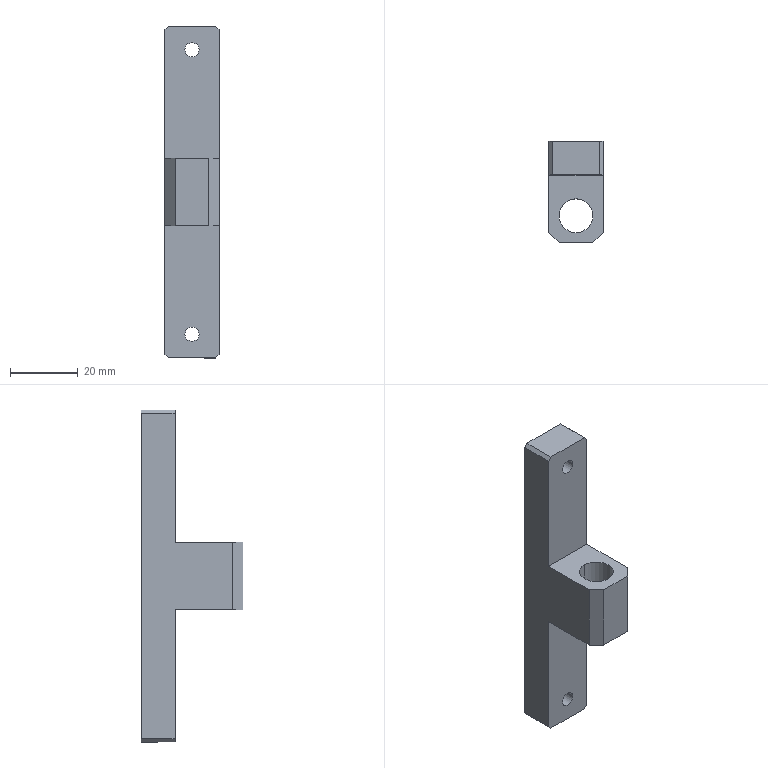Component | SolidWorks | XM-02-007A1-1 | 1 solid | 22 faces | box 16 x 30 x 98 mm | volume 20032 mm3 | plane 16 | cylinder 6 | commonest cylinder face diameters 4.2 x4 10 x2 | material 45#
build123d program:
from build123d import *

# Parameters (mm, degrees)
BOSS_EXTRUDE1_DEPTH = 16
SKETCH2_R           = 5
CUT_EXTRUDE1_DEPTH  = 69.096
M5_TAPPED_HOLE1_D   = 4.2
CHAMFER1_SIZE       = 3
CHAMFER2_SIZE       = 1


with BuildPart() as part:
    # Sketch1 → Boss-Extrude1 (new body)
    with BuildSketch(Plane.XY):
        Polygon((-10, 0), (10, 0), (10, 20), (49, 20), (49, 30), (-49, 30), (-49, 20), (-10, 20), align=None)
    extrude(amount=BOSS_EXTRUDE1_DEPTH)

    # Sketch2 → Cut-Extrude1 (cut, through all)
    with BuildSketch(Plane(origin=(10, 0, 0), x_dir=(0, 0, -1), z_dir=(1, 0, 0))):
        with Locations(Location((-8, 8, 0), (0, 0, 90))):
            Circle(SKETCH2_R)
    extrude(amount=-CUT_EXTRUDE1_DEPTH, mode=Mode.SUBTRACT)

    # M5 Tapped Hole1 (through all)
    with Locations(Plane(origin=(0, 30, 0), x_dir=(1, 0, 0), z_dir=(0, 1, 0))):
        with Locations((42, -8), (-42, -8)):
            Hole(M5_TAPPED_HOLE1_D / 2)

    # Chamfer1
    chamfer1_edges = [part.edges().sort_by_distance(p)[0] for p in [
        (0, 0, 0),
        (0, 0, 16),
    ]]
    chamfer(chamfer1_edges, length=CHAMFER1_SIZE)

    # Chamfer2
    chamfer2_edges = [part.edges().sort_by_distance(p)[0] for p in [
        (49, 25, 16),
        (-49, 25, 16),
        (-49, 25, 0),
        (49, 25, 0),
    ]]
    chamfer(chamfer2_edges, length=CHAMFER2_SIZE)


solid = part.part

# Placed as in the assembly
solid = solid.moved(Location((-5, -33, 0), (0, 90, 0)))
STEP:
#1=COLOUR_RGB('',0.7922,0.8196,0.9333);
#2=FILL_AREA_STYLE_COLOUR('',#1);
#3=FILL_AREA_STYLE('',(#2));
#4=SURFACE_STYLE_FILL_AREA(#3);
#5=SURFACE_SIDE_STYLE('',(#4));
#6=SURFACE_STYLE_USAGE(.BOTH.,#5);
#7=PRESENTATION_STYLE_ASSIGNMENT((#6));
#8=CARTESIAN_POINT('',(0.03543,-0.5118,-1.654));
#9=VERTEX_POINT('',#8);
#10=CARTESIAN_POINT('',(0.2008,-0.5118,-1.654));
#11=VERTEX_POINT('',#10);
#12=CARTESIAN_POINT('',(0.1181,-0.5118,-1.654));
#13=DIRECTION('',(-0.,1.,-0.));
#14=DIRECTION('',(0.,0.,1.));
#15=AXIS2_PLACEMENT_3D('',#12,#13,#14);
#16=CIRCLE('',#15,0.08268);
#17=EDGE_CURVE('',#9,#11,#16,.T.);
#18=ORIENTED_EDGE('',*,*,#17,.F.);
#19=CARTESIAN_POINT('',(0.03543,-0.1181,-1.654));
#20=VERTEX_POINT('',#19);
#21=CARTESIAN_POINT('',(0.03543,-0.1181,-1.654));
#22=DIRECTION('',(-0.,1.,-0.));
#23=VECTOR('',#22,39.37);
#24=LINE('',#21,#23);
#25=EDGE_CURVE('',#9,#20,#24,.T.);
#26=ORIENTED_EDGE('',*,*,#25,.T.);
#27=CARTESIAN_POINT('',(0.2008,-0.1181,-1.654));
#28=VERTEX_POINT('',#27);
#29=CARTESIAN_POINT('',(0.1181,-0.1181,-1.654));
#30=DIRECTION('',(-0.,1.,-0.));
#31=DIRECTION('',(1.,0.,0.));
#32=AXIS2_PLACEMENT_3D('',#29,#30,#31);
#33=CIRCLE('',#32,0.08268);
#34=EDGE_CURVE('',#20,#28,#33,.T.);
#35=ORIENTED_EDGE('',*,*,#34,.T.);
#36=CARTESIAN_POINT('',(0.2008,-0.1181,-1.654));
#37=DIRECTION('',(-0.,1.,-0.));
#38=VECTOR('',#37,39.37);
#39=LINE('',#36,#38);
#40=EDGE_CURVE('',#11,#28,#39,.T.);
#41=ORIENTED_EDGE('',*,*,#40,.F.);
#42=EDGE_LOOP('',(#18,#26,#35,#41));
#43=FACE_OUTER_BOUND('',#42,.T.);
#44=CARTESIAN_POINT('',(0.1181,-0.1181,-1.654));
#45=DIRECTION('',(-0.,1.,-0.));
#46=DIRECTION('',(1.,0.,0.));
#47=AXIS2_PLACEMENT_3D('',#44,#45,#46);
#48=CYLINDRICAL_SURFACE('',#47,0.08268);
#49=ADVANCED_FACE('',(#43),#48,.F.);
#50=CARTESIAN_POINT('',(0.03543,-0.5118,1.654));
#51=VERTEX_POINT('',#50);
#52=CARTESIAN_POINT('',(0.2008,-0.5118,1.654));
#53=VERTEX_POINT('',#52);
#54=CARTESIAN_POINT('',(0.1181,-0.5118,1.654));
#55=DIRECTION('',(-0.,1.,-0.));
#56=DIRECTION('',(0.,0.,1.));
#57=AXIS2_PLACEMENT_3D('',#54,#55,#56);
#58=CIRCLE('',#57,0.08268);
#59=EDGE_CURVE('',#51,#53,#58,.T.);
#60=ORIENTED_EDGE('',*,*,#59,.F.);
#61=CARTESIAN_POINT('',(0.03543,-0.1181,1.654));
#62=VERTEX_POINT('',#61);
#63=CARTESIAN_POINT('',(0.03543,-0.1181,1.654));
#64=DIRECTION('',(-0.,1.,-0.));
#65=VECTOR('',#64,39.37);
#66=LINE('',#63,#65);
#67=EDGE_CURVE('',#51,#62,#66,.T.);
#68=ORIENTED_EDGE('',*,*,#67,.T.);
#69=CARTESIAN_POINT('',(0.2008,-0.1181,1.654));
#70=VERTEX_POINT('',#69);
#71=CARTESIAN_POINT('',(0.1181,-0.1181,1.654));
#72=DIRECTION('',(-0.,1.,-0.));
#73=DIRECTION('',(1.,0.,0.));
#74=AXIS2_PLACEMENT_3D('',#71,#72,#73);
#75=CIRCLE('',#74,0.08268);
#76=EDGE_CURVE('',#62,#70,#75,.T.);
#77=ORIENTED_EDGE('',*,*,#76,.T.);
#78=CARTESIAN_POINT('',(0.2008,-0.1181,1.654));
#79=DIRECTION('',(-0.,1.,-0.));
#80=VECTOR('',#79,39.37);
#81=LINE('',#78,#80);
#82=EDGE_CURVE('',#53,#70,#81,.T.);
#83=ORIENTED_EDGE('',*,*,#82,.F.);
#84=EDGE_LOOP('',(#60,#68,#77,#83));
#85=FACE_OUTER_BOUND('',#84,.T.);
#86=CARTESIAN_POINT('',(0.1181,-0.1181,1.654));
#87=DIRECTION('',(-0.,1.,-0.));
#88=DIRECTION('',(1.,0.,0.));
#89=AXIS2_PLACEMENT_3D('',#86,#87,#88);
#90=CYLINDRICAL_SURFACE('',#89,0.08268);
#91=ADVANCED_FACE('',(#85),#90,.F.);
#92=CARTESIAN_POINT('',(0.1181,-1.181,0.3937));
#93=VERTEX_POINT('',#92);
#94=CARTESIAN_POINT('',(0.1181,-0.7874,0.3937));
#95=VERTEX_POINT('',#94);
#96=CARTESIAN_POINT('',(0.1181,-0.9843,0.3937));
#97=DIRECTION('',(-0.,-0.,-1.));
#98=DIRECTION('',(-1.,0.,0.));
#99=AXIS2_PLACEMENT_3D('',#96,#97,#98);
#100=CIRCLE('',#99,0.1969);
#101=EDGE_CURVE('',#93,#95,#100,.T.);
#102=ORIENTED_EDGE('',*,*,#101,.F.);
#103=CARTESIAN_POINT('',(0.1181,-1.181,-0.3937));
#104=VERTEX_POINT('',#103);
#105=CARTESIAN_POINT('',(0.1181,-1.181,1.929));
#106=DIRECTION('',(-0.,-0.,-1.));
#107=VECTOR('',#106,39.37);
#108=LINE('',#105,#107);
#109=EDGE_CURVE('',#93,#104,#108,.T.);
#110=ORIENTED_EDGE('',*,*,#109,.T.);
#111=CARTESIAN_POINT('',(0.1181,-0.7874,-0.3937));
#112=VERTEX_POINT('',#111);
#113=CARTESIAN_POINT('',(0.1181,-0.9843,-0.3937));
#114=DIRECTION('',(-0.,-0.,-1.));
#115=DIRECTION('',(-0.,1.,-0.));
#116=AXIS2_PLACEMENT_3D('',#113,#114,#115);
#117=CIRCLE('',#116,0.1969);
#118=EDGE_CURVE('',#104,#112,#117,.T.);
#119=ORIENTED_EDGE('',*,*,#118,.T.);
#120=CARTESIAN_POINT('',(0.1181,-0.7874,1.929));
#121=DIRECTION('',(-0.,-0.,-1.));
#122=VECTOR('',#121,39.37);
#123=LINE('',#120,#122);
#124=EDGE_CURVE('',#95,#112,#123,.T.);
#125=ORIENTED_EDGE('',*,*,#124,.F.);
#126=EDGE_LOOP('',(#102,#110,#119,#125));
#127=FACE_OUTER_BOUND('',#126,.T.);
#128=CARTESIAN_POINT('',(0.1181,-0.9843,1.929));
#129=DIRECTION('',(-0.,-0.,-1.));
#130=DIRECTION('',(-0.,1.,-0.));
#131=AXIS2_PLACEMENT_3D('',#128,#129,#130);
#132=CYLINDRICAL_SURFACE('',#131,0.1969);
#133=ADVANCED_FACE('',(#127),#132,.F.);
#134=CARTESIAN_POINT('',(0.1181,-0.9843,0.3937));
#135=DIRECTION('',(-0.,-0.,-1.));
#136=DIRECTION('',(-1.,0.,0.));
#137=AXIS2_PLACEMENT_3D('',#134,#135,#136);
#138=CIRCLE('',#137,0.1969);
#139=EDGE_CURVE('',#95,#93,#138,.T.);
#140=ORIENTED_EDGE('',*,*,#139,.T.);
#141=ORIENTED_EDGE('',*,*,#101,.T.);
#142=EDGE_LOOP('',(#140,#141));
#143=FACE_BOUND('',#142,.T.);
#144=CARTESIAN_POINT('',(0.315,-1.299,0.3937));
#145=VERTEX_POINT('',#144);
#146=CARTESIAN_POINT('',(-0.07874,-1.299,0.3937));
#147=VERTEX_POINT('',#146);
#148=CARTESIAN_POINT('',(0.4331,-1.299,0.3937));
#149=DIRECTION('',(-1.,-0.,0.));
#150=VECTOR('',#149,39.37);
#151=LINE('',#148,#150);
#152=EDGE_CURVE('',#145,#147,#151,.T.);
#153=ORIENTED_EDGE('',*,*,#152,.F.);
#154=CARTESIAN_POINT('',(0.4331,-1.181,0.3937));
#155=VERTEX_POINT('',#154);
#156=CARTESIAN_POINT('',(0.4331,-1.181,0.3937));
#157=DIRECTION('',(0.7071,0.7071,-0.));
#158=VECTOR('',#157,39.37);
#159=LINE('',#156,#158);
#160=EDGE_CURVE('',#145,#155,#159,.T.);
#161=ORIENTED_EDGE('',*,*,#160,.T.);
#162=CARTESIAN_POINT('',(0.4331,-0.5118,0.3937));
#163=VERTEX_POINT('',#162);
#164=CARTESIAN_POINT('',(0.4331,-0.5118,0.3937));
#165=DIRECTION('',(0.,-1.,0.));
#166=VECTOR('',#165,39.37);
#167=LINE('',#164,#166);
#168=EDGE_CURVE('',#163,#155,#167,.T.);
#169=ORIENTED_EDGE('',*,*,#168,.F.);
#170=CARTESIAN_POINT('',(-0.1969,-0.5118,0.3937));
#171=VERTEX_POINT('',#170);
#172=CARTESIAN_POINT('',(0.4331,-0.5118,0.3937));
#173=DIRECTION('',(-1.,-0.,0.));
#174=VECTOR('',#173,39.37);
#175=LINE('',#172,#174);
#176=EDGE_CURVE('',#163,#171,#175,.T.);
#177=ORIENTED_EDGE('',*,*,#176,.T.);
#178=CARTESIAN_POINT('',(-0.1969,-1.181,0.3937));
#179=VERTEX_POINT('',#178);
#180=CARTESIAN_POINT('',(-0.1969,-0.5118,0.3937));
#181=DIRECTION('',(0.,-1.,0.));
#182=VECTOR('',#181,39.37);
#183=LINE('',#180,#182);
#184=EDGE_CURVE('',#171,#179,#183,.T.);
#185=ORIENTED_EDGE('',*,*,#184,.T.);
#186=CARTESIAN_POINT('',(-0.07874,-1.299,0.3937));
#187=DIRECTION('',(0.7071,-0.7071,0.));
#188=VECTOR('',#187,39.37);
#189=LINE('',#186,#188);
#190=EDGE_CURVE('',#179,#147,#189,.T.);
#191=ORIENTED_EDGE('',*,*,#190,.T.);
#192=EDGE_LOOP('',(#153,#161,#169,#177,#185,#191));
#193=FACE_OUTER_BOUND('',#192,.T.);
#194=CARTESIAN_POINT('',(0.4331,-0.5118,0.3937));
#195=DIRECTION('',(-0.,-0.,-1.));
#196=DIRECTION('',(-1.,-0.,0.));
#197=AXIS2_PLACEMENT_3D('',#194,#195,#196);
#198=PLANE('',#197);
#199=ADVANCED_FACE('',(#143,#193),#198,.F.);
#200=CARTESIAN_POINT('',(0.315,-1.299,-0.3937));
#201=VERTEX_POINT('',#200);
#202=CARTESIAN_POINT('',(-0.07874,-1.299,-0.3937));
#203=VERTEX_POINT('',#202);
#204=CARTESIAN_POINT('',(0.4331,-1.299,-0.3937));
#205=DIRECTION('',(-1.,-0.,0.));
#206=VECTOR('',#205,39.37);
#207=LINE('',#204,#206);
#208=EDGE_CURVE('',#201,#203,#207,.T.);
#209=ORIENTED_EDGE('',*,*,#208,.F.);
#210=CARTESIAN_POINT('',(0.315,-1.299,0.3937));
#211=DIRECTION('',(0.,0.,1.));
#212=VECTOR('',#211,39.37);
#213=LINE('',#210,#212);
#214=EDGE_CURVE('',#201,#145,#213,.T.);
#215=ORIENTED_EDGE('',*,*,#214,.T.);
#216=ORIENTED_EDGE('',*,*,#152,.T.);
#217=CARTESIAN_POINT('',(-0.07874,-1.299,0.3937));
#218=DIRECTION('',(-0.,-0.,-1.));
#219=VECTOR('',#218,39.37);
#220=LINE('',#217,#219);
#221=EDGE_CURVE('',#147,#203,#220,.T.);
#222=ORIENTED_EDGE('',*,*,#221,.T.);
#223=EDGE_LOOP('',(#209,#215,#216,#222));
#224=FACE_OUTER_BOUND('',#223,.T.);
#225=CARTESIAN_POINT('',(0.4331,-1.299,0.3937));
#226=DIRECTION('',(-0.,1.,-0.));
#227=DIRECTION('',(0.,0.,1.));
#228=AXIS2_PLACEMENT_3D('',#225,#226,#227);
#229=PLANE('',#228);
#230=ADVANCED_FACE('',(#224),#229,.F.);
#231=CARTESIAN_POINT('',(0.1181,-0.9843,-0.3937));
#232=DIRECTION('',(-0.,-0.,-1.));
#233=DIRECTION('',(-0.,1.,-0.));
#234=AXIS2_PLACEMENT_3D('',#231,#232,#233);
#235=CIRCLE('',#234,0.1969);
#236=EDGE_CURVE('',#112,#104,#235,.T.);
#237=ORIENTED_EDGE('',*,*,#236,.F.);
#238=ORIENTED_EDGE('',*,*,#118,.F.);
#239=EDGE_LOOP('',(#237,#238));
#240=FACE_BOUND('',#239,.T.);
#241=CARTESIAN_POINT('',(0.4331,-1.181,-0.3937));
#242=VERTEX_POINT('',#241);
#243=CARTESIAN_POINT('',(0.4331,-0.5118,-0.3937));
#244=VERTEX_POINT('',#243);
#245=CARTESIAN_POINT('',(0.4331,-1.299,-0.3937));
#246=DIRECTION('',(-0.,1.,-0.));
#247=VECTOR('',#246,39.37);
#248=LINE('',#245,#247);
#249=EDGE_CURVE('',#242,#244,#248,.T.);
#250=ORIENTED_EDGE('',*,*,#249,.F.);
#251=CARTESIAN_POINT('',(0.4331,-1.181,-0.3937));
#252=DIRECTION('',(-0.7071,-0.7071,0.));
#253=VECTOR('',#252,39.37);
#254=LINE('',#251,#253);
#255=EDGE_CURVE('',#242,#201,#254,.T.);
#256=ORIENTED_EDGE('',*,*,#255,.T.);
#257=ORIENTED_EDGE('',*,*,#208,.T.);
#258=CARTESIAN_POINT('',(-0.1969,-1.181,-0.3937));
#259=VERTEX_POINT('',#258);
#260=CARTESIAN_POINT('',(-0.07874,-1.299,-0.3937));
#261=DIRECTION('',(-0.7071,0.7071,-0.));
#262=VECTOR('',#261,39.37);
#263=LINE('',#260,#262);
#264=EDGE_CURVE('',#203,#259,#263,.T.);
#265=ORIENTED_EDGE('',*,*,#264,.T.);
#266=CARTESIAN_POINT('',(-0.1969,-0.5118,-0.3937));
#267=VERTEX_POINT('',#266);
#268=CARTESIAN_POINT('',(-0.1969,-1.299,-0.3937));
#269=DIRECTION('',(-0.,1.,-0.));
#270=VECTOR('',#269,39.37);
#271=LINE('',#268,#270);
#272=EDGE_CURVE('',#259,#267,#271,.T.);
#273=ORIENTED_EDGE('',*,*,#272,.T.);
#274=CARTESIAN_POINT('',(0.4331,-0.5118,-0.3937));
#275=DIRECTION('',(-1.,-0.,0.));
#276=VECTOR('',#275,39.37);
#277=LINE('',#274,#276);
#278=EDGE_CURVE('',#244,#267,#277,.T.);
#279=ORIENTED_EDGE('',*,*,#278,.F.);
#280=EDGE_LOOP('',(#250,#256,#257,#265,#273,#279));
#281=FACE_OUTER_BOUND('',#280,.T.);
#282=CARTESIAN_POINT('',(0.4331,-1.299,-0.3937));
#283=DIRECTION('',(0.,0.,1.));
#284=DIRECTION('',(0.,-1.,0.));
#285=AXIS2_PLACEMENT_3D('',#282,#283,#284);
#286=PLANE('',#285);
#287=ADVANCED_FACE('',(#240,#281),#286,.F.);
#288=CARTESIAN_POINT('',(0.1181,-0.5118,-1.654));
#289=DIRECTION('',(-0.,1.,-0.));
#290=DIRECTION('',(0.,0.,1.));
#291=AXIS2_PLACEMENT_3D('',#288,#289,#290);
#292=CIRCLE('',#291,0.08268);
#293=EDGE_CURVE('',#11,#9,#292,.T.);
#294=ORIENTED_EDGE('',*,*,#293,.T.);
#295=ORIENTED_EDGE('',*,*,#17,.T.);
#296=EDGE_LOOP('',(#294,#295));
#297=FACE_BOUND('',#296,.T.);
#298=CARTESIAN_POINT('',(0.3937,-0.5118,-1.929));
#299=VERTEX_POINT('',#298);
#300=CARTESIAN_POINT('',(-0.1575,-0.5118,-1.929));
#301=VERTEX_POINT('',#300);
#302=CARTESIAN_POINT('',(0.4331,-0.5118,-1.929));
#303=DIRECTION('',(-1.,-0.,0.));
#304=VECTOR('',#303,39.37);
#305=LINE('',#302,#304);
#306=EDGE_CURVE('',#299,#301,#305,.T.);
#307=ORIENTED_EDGE('',*,*,#306,.F.);
#308=CARTESIAN_POINT('',(0.4331,-0.5118,-1.89));
#309=VERTEX_POINT('',#308);
#310=CARTESIAN_POINT('',(0.4331,-0.5118,-1.89));
#311=DIRECTION('',(0.7071,0.,0.7071));
#312=VECTOR('',#311,39.37);
#313=LINE('',#310,#312);
#314=EDGE_CURVE('',#299,#309,#313,.T.);
#315=ORIENTED_EDGE('',*,*,#314,.T.);
#316=CARTESIAN_POINT('',(0.4331,-0.5118,-0.3937));
#317=DIRECTION('',(-0.,-0.,-1.));
#318=VECTOR('',#317,39.37);
#319=LINE('',#316,#318);
#320=EDGE_CURVE('',#244,#309,#319,.T.);
#321=ORIENTED_EDGE('',*,*,#320,.F.);
#322=ORIENTED_EDGE('',*,*,#278,.T.);
#323=CARTESIAN_POINT('',(-0.1969,-0.5118,-1.89));
#324=VERTEX_POINT('',#323);
#325=CARTESIAN_POINT('',(-0.1969,-0.5118,-0.3937));
#326=DIRECTION('',(-0.,-0.,-1.));
#327=VECTOR('',#326,39.37);
#328=LINE('',#325,#327);
#329=EDGE_CURVE('',#267,#324,#328,.T.);
#330=ORIENTED_EDGE('',*,*,#329,.T.);
#331=CARTESIAN_POINT('',(-0.1575,-0.5118,-1.929));
#332=DIRECTION('',(0.7071,-0.,-0.7071));
#333=VECTOR('',#332,39.37);
#334=LINE('',#331,#333);
#335=EDGE_CURVE('',#324,#301,#334,.T.);
#336=ORIENTED_EDGE('',*,*,#335,.T.);
#337=EDGE_LOOP('',(#307,#315,#321,#322,#330,#336));
#338=FACE_OUTER_BOUND('',#337,.T.);
#339=CARTESIAN_POINT('',(0.4331,-0.5118,-0.3937));
#340=DIRECTION('',(-0.,1.,-0.));
#341=DIRECTION('',(0.,0.,1.));
#342=AXIS2_PLACEMENT_3D('',#339,#340,#341);
#343=PLANE('',#342);
#344=ADVANCED_FACE('',(#297,#338),#343,.F.);
#345=CARTESIAN_POINT('',(0.3937,-0.1181,-1.929));
#346=VERTEX_POINT('',#345);
#347=CARTESIAN_POINT('',(-0.1575,-0.1181,-1.929));
#348=VERTEX_POINT('',#347);
#349=CARTESIAN_POINT('',(0.4331,-0.1181,-1.929));
#350=DIRECTION('',(-1.,-0.,0.));
#351=VECTOR('',#350,39.37);
#352=LINE('',#349,#351);
#353=EDGE_CURVE('',#346,#348,#352,.T.);
#354=ORIENTED_EDGE('',*,*,#353,.F.);
#355=CARTESIAN_POINT('',(0.3937,-0.5118,-1.929));
#356=DIRECTION('',(0.,-1.,0.));
#357=VECTOR('',#356,39.37);
#358=LINE('',#355,#357);
#359=EDGE_CURVE('',#346,#299,#358,.T.);
#360=ORIENTED_EDGE('',*,*,#359,.T.);
#361=ORIENTED_EDGE('',*,*,#306,.T.);
#362=CARTESIAN_POINT('',(-0.1575,-0.5118,-1.929));
#363=DIRECTION('',(-0.,1.,-0.));
#364=VECTOR('',#363,39.37);
#365=LINE('',#362,#364);
#366=EDGE_CURVE('',#301,#348,#365,.T.);
#367=ORIENTED_EDGE('',*,*,#366,.T.);
#368=EDGE_LOOP('',(#354,#360,#361,#367));
#369=FACE_OUTER_BOUND('',#368,.T.);
#370=CARTESIAN_POINT('',(0.4331,-0.5118,-1.929));
#371=DIRECTION('',(0.,0.,1.));
#372=DIRECTION('',(1.,0.,-0.));
#373=AXIS2_PLACEMENT_3D('',#370,#371,#372);
#374=PLANE('',#373);
#375=ADVANCED_FACE('',(#369),#374,.F.);
#376=CARTESIAN_POINT('',(0.1181,-0.1181,-1.654));
#377=DIRECTION('',(-0.,1.,-0.));
#378=DIRECTION('',(1.,0.,0.));
#379=AXIS2_PLACEMENT_3D('',#376,#377,#378);
#380=CIRCLE('',#379,0.08268);
#381=EDGE_CURVE('',#28,#20,#380,.T.);
#382=ORIENTED_EDGE('',*,*,#381,.F.);
#383=ORIENTED_EDGE('',*,*,#34,.F.);
#384=EDGE_LOOP('',(#382,#383));
#385=FACE_BOUND('',#384,.T.);
#386=CARTESIAN_POINT('',(0.1181,-0.1181,1.654));
#387=DIRECTION('',(-0.,1.,-0.));
#388=DIRECTION('',(1.,0.,0.));
#389=AXIS2_PLACEMENT_3D('',#386,#387,#388);
#390=CIRCLE('',#389,0.08268);
#391=EDGE_CURVE('',#70,#62,#390,.T.);
#392=ORIENTED_EDGE('',*,*,#391,.F.);
#393=ORIENTED_EDGE('',*,*,#76,.F.);
#394=EDGE_LOOP('',(#392,#393));
#395=FACE_BOUND('',#394,.T.);
#396=CARTESIAN_POINT('',(0.4331,-0.1181,-1.89));
#397=VERTEX_POINT('',#396);
#398=CARTESIAN_POINT('',(0.4331,-0.1181,1.89));
#399=VERTEX_POINT('',#398);
#400=CARTESIAN_POINT('',(0.4331,-0.1181,-1.929));
#401=DIRECTION('',(0.,0.,1.));
#402=VECTOR('',#401,39.37);
#403=LINE('',#400,#402);
#404=EDGE_CURVE('',#397,#399,#403,.T.);
#405=ORIENTED_EDGE('',*,*,#404,.F.);
#406=CARTESIAN_POINT('',(0.4331,-0.1181,-1.89));
#407=DIRECTION('',(-0.7071,-0.,-0.7071));
#408=VECTOR('',#407,39.37);
#409=LINE('',#406,#408);
#410=EDGE_CURVE('',#397,#346,#409,.T.);
#411=ORIENTED_EDGE('',*,*,#410,.T.);
#412=ORIENTED_EDGE('',*,*,#353,.T.);
#413=CARTESIAN_POINT('',(-0.1969,-0.1181,-1.89));
#414=VERTEX_POINT('',#413);
#415=CARTESIAN_POINT('',(-0.1575,-0.1181,-1.929));
#416=DIRECTION('',(-0.7071,0.,0.7071));
#417=VECTOR('',#416,39.37);
#418=LINE('',#415,#417);
#419=EDGE_CURVE('',#348,#414,#418,.T.);
#420=ORIENTED_EDGE('',*,*,#419,.T.);
#421=CARTESIAN_POINT('',(-0.1969,-0.1181,1.89));
#422=VERTEX_POINT('',#421);
#423=CARTESIAN_POINT('',(-0.1969,-0.1181,-1.929));
#424=DIRECTION('',(0.,0.,1.));
#425=VECTOR('',#424,39.37);
#426=LINE('',#423,#425);
#427=EDGE_CURVE('',#414,#422,#426,.T.);
#428=ORIENTED_EDGE('',*,*,#427,.T.);
#429=CARTESIAN_POINT('',(-0.1575,-0.1181,1.929));
#430=VERTEX_POINT('',#429);
#431=CARTESIAN_POINT('',(-0.1575,-0.1181,1.929));
#432=DIRECTION('',(0.7071,0.,0.7071));
#433=VECTOR('',#432,39.37);
#434=LINE('',#431,#433);
#435=EDGE_CURVE('',#422,#430,#434,.T.);
#436=ORIENTED_EDGE('',*,*,#435,.T.);
#437=CARTESIAN_POINT('',(0.3937,-0.1181,1.929));
#438=VERTEX_POINT('',#437);
#439=CARTESIAN_POINT('',(0.4331,-0.1181,1.929));
#440=DIRECTION('',(-1.,-0.,0.));
#441=VECTOR('',#440,39.37);
#442=LINE('',#439,#441);
#443=EDGE_CURVE('',#438,#430,#442,.T.);
#444=ORIENTED_EDGE('',*,*,#443,.F.);
#445=CARTESIAN_POINT('',(0.4331,-0.1181,1.89));
#446=DIRECTION('',(0.7071,-0.,-0.7071));
#447=VECTOR('',#446,39.37);
#448=LINE('',#445,#447);
#449=EDGE_CURVE('',#438,#399,#448,.T.);
#450=ORIENTED_EDGE('',*,*,#449,.T.);
#451=EDGE_LOOP('',(#405,#411,#412,#420,#428,#436,#444,#450));
#452=FACE_OUTER_BOUND('',#451,.T.);
#453=CARTESIAN_POINT('',(0.4331,-0.1181,-1.929));
#454=DIRECTION('',(0.,-1.,0.));
#455=DIRECTION('',(-0.,-0.,-1.));
#456=AXIS2_PLACEMENT_3D('',#453,#454,#455);
#457=PLANE('',#456);
#458=ADVANCED_FACE('',(#385,#395,#452),#457,.F.);
#459=CARTESIAN_POINT('',(0.3937,-0.5118,1.929));
#460=VERTEX_POINT('',#459);
#461=CARTESIAN_POINT('',(-0.1575,-0.5118,1.929));
#462=VERTEX_POINT('',#461);
#463=CARTESIAN_POINT('',(0.4331,-0.5118,1.929));
#464=DIRECTION('',(-1.,-0.,0.));
#465=VECTOR('',#464,39.37);
#466=LINE('',#463,#465);
#467=EDGE_CURVE('',#460,#462,#466,.T.);
#468=ORIENTED_EDGE('',*,*,#467,.F.);
#469=CARTESIAN_POINT('',(0.3937,-0.1181,1.929));
#470=DIRECTION('',(-0.,1.,-0.));
#471=VECTOR('',#470,39.37);
#472=LINE('',#469,#471);
#473=EDGE_CURVE('',#460,#438,#472,.T.);
#474=ORIENTED_EDGE('',*,*,#473,.T.);
#475=ORIENTED_EDGE('',*,*,#443,.T.);
#476=CARTESIAN_POINT('',(-0.1575,-0.1181,1.929));
#477=DIRECTION('',(0.,-1.,0.));
#478=VECTOR('',#477,39.37);
#479=LINE('',#476,#478);
#480=EDGE_CURVE('',#430,#462,#479,.T.);
#481=ORIENTED_EDGE('',*,*,#480,.T.);
#482=EDGE_LOOP('',(#468,#474,#475,#481));
#483=FACE_OUTER_BOUND('',#482,.T.);
#484=CARTESIAN_POINT('',(0.4331,-0.1181,1.929));
#485=DIRECTION('',(-0.,-0.,-1.));
#486=DIRECTION('',(-0.,1.,-0.));
#487=AXIS2_PLACEMENT_3D('',#484,#485,#486);
#488=PLANE('',#487);
#489=ADVANCED_FACE('',(#483),#488,.F.);
#490=CARTESIAN_POINT('',(0.1181,-0.5118,1.654));
#491=DIRECTION('',(-0.,1.,-0.));
#492=DIRECTION('',(0.,0.,1.));
#493=AXIS2_PLACEMENT_3D('',#490,#491,#492);
#494=CIRCLE('',#493,0.08268);
#495=EDGE_CURVE('',#53,#51,#494,.T.);
#496=ORIENTED_EDGE('',*,*,#495,.T.);
#497=ORIENTED_EDGE('',*,*,#59,.T.);
#498=EDGE_LOOP('',(#496,#497));
#499=FACE_BOUND('',#498,.T.);
#500=CARTESIAN_POINT('',(0.4331,-0.5118,1.89));
#501=VERTEX_POINT('',#500);
#502=CARTESIAN_POINT('',(0.4331,-0.5118,1.929));
#503=DIRECTION('',(-0.,-0.,-1.));
#504=VECTOR('',#503,39.37);
#505=LINE('',#502,#504);
#506=EDGE_CURVE('',#501,#163,#505,.T.);
#507=ORIENTED_EDGE('',*,*,#506,.F.);
#508=CARTESIAN_POINT('',(0.4331,-0.5118,1.89));
#509=DIRECTION('',(-0.7071,0.,0.7071));
#510=VECTOR('',#509,39.37);
#511=LINE('',#508,#510);
#512=EDGE_CURVE('',#501,#460,#511,.T.);
#513=ORIENTED_EDGE('',*,*,#512,.T.);
#514=ORIENTED_EDGE('',*,*,#467,.T.);
#515=CARTESIAN_POINT('',(-0.1969,-0.5118,1.89));
#516=VERTEX_POINT('',#515);
#517=CARTESIAN_POINT('',(-0.1575,-0.5118,1.929));
#518=DIRECTION('',(-0.7071,-0.,-0.7071));
#519=VECTOR('',#518,39.37);
#520=LINE('',#517,#519);
#521=EDGE_CURVE('',#462,#516,#520,.T.);
#522=ORIENTED_EDGE('',*,*,#521,.T.);
#523=CARTESIAN_POINT('',(-0.1969,-0.5118,1.929));
#524=DIRECTION('',(-0.,-0.,-1.));
#525=VECTOR('',#524,39.37);
#526=LINE('',#523,#525);
#527=EDGE_CURVE('',#516,#171,#526,.T.);
#528=ORIENTED_EDGE('',*,*,#527,.T.);
#529=ORIENTED_EDGE('',*,*,#176,.F.);
#530=EDGE_LOOP('',(#507,#513,#514,#522,#528,#529));
#531=FACE_OUTER_BOUND('',#530,.T.);
#532=CARTESIAN_POINT('',(0.4331,-0.5118,1.929));
#533=DIRECTION('',(-0.,1.,-0.));
#534=DIRECTION('',(0.,0.,1.));
#535=AXIS2_PLACEMENT_3D('',#532,#533,#534);
#536=PLANE('',#535);
#537=ADVANCED_FACE('',(#499,#531),#536,.F.);
#538=ORIENTED_EDGE('',*,*,#320,.T.);
#539=CARTESIAN_POINT('',(0.4331,-0.1181,-1.89));
#540=DIRECTION('',(-0.,1.,-0.));
#541=VECTOR('',#540,39.37);
#542=LINE('',#539,#541);
#543=EDGE_CURVE('',#309,#397,#542,.T.);
#544=ORIENTED_EDGE('',*,*,#543,.T.);
#545=ORIENTED_EDGE('',*,*,#404,.T.);
#546=CARTESIAN_POINT('',(0.4331,-0.5118,1.89));
#547=DIRECTION('',(0.,-1.,0.));
#548=VECTOR('',#547,39.37);
#549=LINE('',#546,#548);
#550=EDGE_CURVE('',#399,#501,#549,.T.);
#551=ORIENTED_EDGE('',*,*,#550,.T.);
#552=ORIENTED_EDGE('',*,*,#506,.T.);
#553=ORIENTED_EDGE('',*,*,#168,.T.);
#554=CARTESIAN_POINT('',(0.4331,-1.181,-0.3937));
#555=DIRECTION('',(-0.,-0.,-1.));
#556=VECTOR('',#555,39.37);
#557=LINE('',#554,#556);
#558=EDGE_CURVE('',#155,#242,#557,.T.);
#559=ORIENTED_EDGE('',*,*,#558,.T.);
#560=ORIENTED_EDGE('',*,*,#249,.T.);
#561=EDGE_LOOP('',(#538,#544,#545,#551,#552,#553,#559,#560));
#562=FACE_OUTER_BOUND('',#561,.T.);
#563=CARTESIAN_POINT('',(0.4331,-1.299,0.));
#564=DIRECTION('',(1.,0.,-0.));
#565=DIRECTION('',(-0.,-0.,-1.));
#566=AXIS2_PLACEMENT_3D('',#563,#564,#565);
#567=PLANE('',#566);
#568=ADVANCED_FACE('',(#562),#567,.T.);
#569=ORIENTED_EDGE('',*,*,#427,.F.);
#570=CARTESIAN_POINT('',(-0.1969,-1.299,-1.89));
#571=DIRECTION('',(0.,-1.,0.));
#572=VECTOR('',#571,39.37);
#573=LINE('',#570,#572);
#574=EDGE_CURVE('',#414,#324,#573,.T.);
#575=ORIENTED_EDGE('',*,*,#574,.T.);
#576=ORIENTED_EDGE('',*,*,#329,.F.);
#577=ORIENTED_EDGE('',*,*,#272,.F.);
#578=CARTESIAN_POINT('',(-0.1969,-1.181,0.));
#579=DIRECTION('',(0.,0.,1.));
#580=VECTOR('',#579,39.37);
#581=LINE('',#578,#580);
#582=EDGE_CURVE('',#259,#179,#581,.T.);
#583=ORIENTED_EDGE('',*,*,#582,.T.);
#584=ORIENTED_EDGE('',*,*,#184,.F.);
#585=ORIENTED_EDGE('',*,*,#527,.F.);
#586=CARTESIAN_POINT('',(-0.1969,-1.299,1.89));
#587=DIRECTION('',(-0.,1.,-0.));
#588=VECTOR('',#587,39.37);
#589=LINE('',#586,#588);
#590=EDGE_CURVE('',#516,#422,#589,.T.);
#591=ORIENTED_EDGE('',*,*,#590,.T.);
#592=EDGE_LOOP('',(#569,#575,#576,#577,#583,#584,#585,#591));
#593=FACE_OUTER_BOUND('',#592,.T.);
#594=CARTESIAN_POINT('',(-0.1969,-1.299,0.));
#595=DIRECTION('',(1.,0.,-0.));
#596=DIRECTION('',(-0.,-0.,-1.));
#597=AXIS2_PLACEMENT_3D('',#594,#595,#596);
#598=PLANE('',#597);
#599=ADVANCED_FACE('',(#593),#598,.F.);
#600=ORIENTED_EDGE('',*,*,#109,.F.);
#601=ORIENTED_EDGE('',*,*,#139,.F.);
#602=ORIENTED_EDGE('',*,*,#124,.T.);
#603=ORIENTED_EDGE('',*,*,#236,.T.);
#604=EDGE_LOOP('',(#600,#601,#602,#603));
#605=FACE_OUTER_BOUND('',#604,.T.);
#606=CARTESIAN_POINT('',(0.1181,-0.9843,1.929));
#607=DIRECTION('',(-0.,-0.,-1.));
#608=DIRECTION('',(-0.,1.,-0.));
#609=AXIS2_PLACEMENT_3D('',#606,#607,#608);
#610=CYLINDRICAL_SURFACE('',#609,0.1969);
#611=ADVANCED_FACE('',(#605),#610,.F.);
#612=ORIENTED_EDGE('',*,*,#67,.F.);
#613=ORIENTED_EDGE('',*,*,#495,.F.);
#614=ORIENTED_EDGE('',*,*,#82,.T.);
#615=ORIENTED_EDGE('',*,*,#391,.T.);
#616=EDGE_LOOP('',(#612,#613,#614,#615));
#617=FACE_OUTER_BOUND('',#616,.T.);
#618=CARTESIAN_POINT('',(0.1181,-0.1181,1.654));
#619=DIRECTION('',(-0.,1.,-0.));
#620=DIRECTION('',(1.,0.,0.));
#621=AXIS2_PLACEMENT_3D('',#618,#619,#620);
#622=CYLINDRICAL_SURFACE('',#621,0.08268);
#623=ADVANCED_FACE('',(#617),#622,.F.);
#624=ORIENTED_EDGE('',*,*,#25,.F.);
#625=ORIENTED_EDGE('',*,*,#293,.F.);
#626=ORIENTED_EDGE('',*,*,#40,.T.);
#627=ORIENTED_EDGE('',*,*,#381,.T.);
#628=EDGE_LOOP('',(#624,#625,#626,#627));
#629=FACE_OUTER_BOUND('',#628,.T.);
#630=CARTESIAN_POINT('',(0.1181,-0.1181,-1.654));
#631=DIRECTION('',(-0.,1.,-0.));
#632=DIRECTION('',(1.,0.,0.));
#633=AXIS2_PLACEMENT_3D('',#630,#631,#632);
#634=CYLINDRICAL_SURFACE('',#633,0.08268);
#635=ADVANCED_FACE('',(#629),#634,.F.);
#636=ORIENTED_EDGE('',*,*,#160,.F.);
#637=ORIENTED_EDGE('',*,*,#214,.F.);
#638=ORIENTED_EDGE('',*,*,#255,.F.);
#639=ORIENTED_EDGE('',*,*,#558,.F.);
#640=EDGE_LOOP('',(#636,#637,#638,#639));
#641=FACE_OUTER_BOUND('',#640,.T.);
#642=CARTESIAN_POINT('',(0.4331,-1.181,0.));
#643=DIRECTION('',(0.7071,-0.7071,0.));
#644=DIRECTION('',(0.,0.,1.));
#645=AXIS2_PLACEMENT_3D('',#642,#643,#644);
#646=PLANE('',#645);
#647=ADVANCED_FACE('',(#641),#646,.T.);
#648=ORIENTED_EDGE('',*,*,#190,.F.);
#649=ORIENTED_EDGE('',*,*,#582,.F.);
#650=ORIENTED_EDGE('',*,*,#264,.F.);
#651=ORIENTED_EDGE('',*,*,#221,.F.);
#652=EDGE_LOOP('',(#648,#649,#650,#651));
#653=FACE_OUTER_BOUND('',#652,.T.);
#654=CARTESIAN_POINT('',(-0.07874,-1.299,0.3937));
#655=DIRECTION('',(0.7071,0.7071,-0.));
#656=DIRECTION('',(-0.,-0.,-1.));
#657=AXIS2_PLACEMENT_3D('',#654,#655,#656);
#658=PLANE('',#657);
#659=ADVANCED_FACE('',(#653),#658,.F.);
#660=ORIENTED_EDGE('',*,*,#314,.F.);
#661=ORIENTED_EDGE('',*,*,#359,.F.);
#662=ORIENTED_EDGE('',*,*,#410,.F.);
#663=ORIENTED_EDGE('',*,*,#543,.F.);
#664=EDGE_LOOP('',(#660,#661,#662,#663));
#665=FACE_OUTER_BOUND('',#664,.T.);
#666=CARTESIAN_POINT('',(0.4331,-1.299,-1.89));
#667=DIRECTION('',(0.7071,-0.,-0.7071));
#668=DIRECTION('',(0.,-1.,0.));
#669=AXIS2_PLACEMENT_3D('',#666,#667,#668);
#670=PLANE('',#669);
#671=ADVANCED_FACE('',(#665),#670,.T.);
#672=ORIENTED_EDGE('',*,*,#335,.F.);
#673=ORIENTED_EDGE('',*,*,#574,.F.);
#674=ORIENTED_EDGE('',*,*,#419,.F.);
#675=ORIENTED_EDGE('',*,*,#366,.F.);
#676=EDGE_LOOP('',(#672,#673,#674,#675));
#677=FACE_OUTER_BOUND('',#676,.T.);
#678=CARTESIAN_POINT('',(-0.1575,-0.5118,-1.929));
#679=DIRECTION('',(0.7071,0.,0.7071));
#680=DIRECTION('',(-0.,1.,-0.));
#681=AXIS2_PLACEMENT_3D('',#678,#679,#680);
#682=PLANE('',#681);
#683=ADVANCED_FACE('',(#677),#682,.F.);
#684=ORIENTED_EDGE('',*,*,#449,.F.);
#685=ORIENTED_EDGE('',*,*,#473,.F.);
#686=ORIENTED_EDGE('',*,*,#512,.F.);
#687=ORIENTED_EDGE('',*,*,#550,.F.);
#688=EDGE_LOOP('',(#684,#685,#686,#687));
#689=FACE_OUTER_BOUND('',#688,.T.);
#690=CARTESIAN_POINT('',(0.4331,-1.299,1.89));
#691=DIRECTION('',(0.7071,0.,0.7071));
#692=DIRECTION('',(-0.,1.,-0.));
#693=AXIS2_PLACEMENT_3D('',#690,#691,#692);
#694=PLANE('',#693);
#695=ADVANCED_FACE('',(#689),#694,.T.);
#696=ORIENTED_EDGE('',*,*,#435,.F.);
#697=ORIENTED_EDGE('',*,*,#590,.F.);
#698=ORIENTED_EDGE('',*,*,#521,.F.);
#699=ORIENTED_EDGE('',*,*,#480,.F.);
#700=EDGE_LOOP('',(#696,#697,#698,#699));
#701=FACE_OUTER_BOUND('',#700,.T.);
#702=CARTESIAN_POINT('',(-0.1575,-0.1181,1.929));
#703=DIRECTION('',(0.7071,-0.,-0.7071));
#704=DIRECTION('',(0.,-1.,0.));
#705=AXIS2_PLACEMENT_3D('',#702,#703,#704);
#706=PLANE('',#705);
#707=ADVANCED_FACE('',(#701),#706,.F.);
#708=CLOSED_SHELL('',(#49,#91,#133,#199,#230,#287,#344,#375,#458,#489,#537,#568,#599,#611,#623,#635,#647,#659,#671,#683,#695,#707));
#709=MANIFOLD_SOLID_BREP('',#708);
#710=STYLED_ITEM('',(#7),#709);
#711=(LENGTH_UNIT()NAMED_UNIT(*)SI_UNIT($,.METRE.));
#712=LENGTH_MEASURE_WITH_UNIT(LENGTH_MEASURE(0.0254),#711);
#713=DIMENSIONAL_EXPONENTS(1.,0.,0.,0.,0.,0.,0.);
#714=(CONVERSION_BASED_UNIT('',#712)LENGTH_UNIT()NAMED_UNIT(#713));
#715=UNCERTAINTY_MEASURE_WITH_UNIT(LENGTH_MEASURE(0.00001),#714,'','');
#716=(NAMED_UNIT(*)PLANE_ANGLE_UNIT()SI_UNIT($,.RADIAN.));
#717=(NAMED_UNIT(*)SI_UNIT($,.STERADIAN.)SOLID_ANGLE_UNIT());
#718=(GEOMETRIC_REPRESENTATION_CONTEXT(3)GLOBAL_UNCERTAINTY_ASSIGNED_CONTEXT((#715))GLOBAL_UNIT_ASSIGNED_CONTEXT((#714,#716,#717))REPRESENTATION_CONTEXT('',''));
#719=MECHANICAL_DESIGN_GEOMETRIC_PRESENTATION_REPRESENTATION('',(#710),#718);
#720=PRESENTATION_LAYER_ASSIGNMENT('','',(#710));
#721=CARTESIAN_POINT('',(0.,0.,0.));
#722=DIRECTION('',(0.,0.,1.));
#723=DIRECTION('',(1.,0.,0.));
#724=AXIS2_PLACEMENT_3D('',#721,#722,#723);
#725=(LENGTH_UNIT()NAMED_UNIT(*)SI_UNIT($,.METRE.));
#726=LENGTH_MEASURE_WITH_UNIT(LENGTH_MEASURE(0.0254),#725);
#727=DIMENSIONAL_EXPONENTS(1.,0.,0.,0.,0.,0.,0.);
#728=(CONVERSION_BASED_UNIT('',#726)LENGTH_UNIT()NAMED_UNIT(#727));
#729=UNCERTAINTY_MEASURE_WITH_UNIT(LENGTH_MEASURE(0.00001),#728,'','');
#730=(NAMED_UNIT(*)PLANE_ANGLE_UNIT()SI_UNIT($,.RADIAN.));
#731=(NAMED_UNIT(*)SI_UNIT($,.STERADIAN.)SOLID_ANGLE_UNIT());
#732=(GEOMETRIC_REPRESENTATION_CONTEXT(3)GLOBAL_UNCERTAINTY_ASSIGNED_CONTEXT((#729))GLOBAL_UNIT_ASSIGNED_CONTEXT((#728,#730,#731))REPRESENTATION_CONTEXT('',''));
#733=ADVANCED_BREP_SHAPE_REPRESENTATION('',(#709,#724),#732);